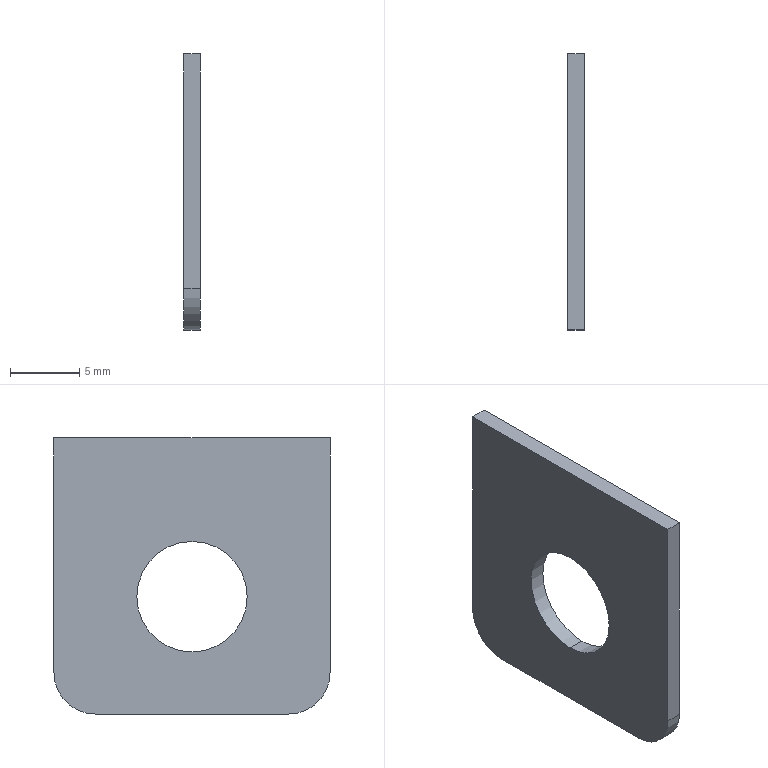Component | SolidWorks | CabinetWelding-1_RearDoorFixingPlate-2 | 1 solid | 10 faces | volume 415 mm3 | plane 6 | cylinder 4 | commonest cylinder face diameters 8 x2 6 x2